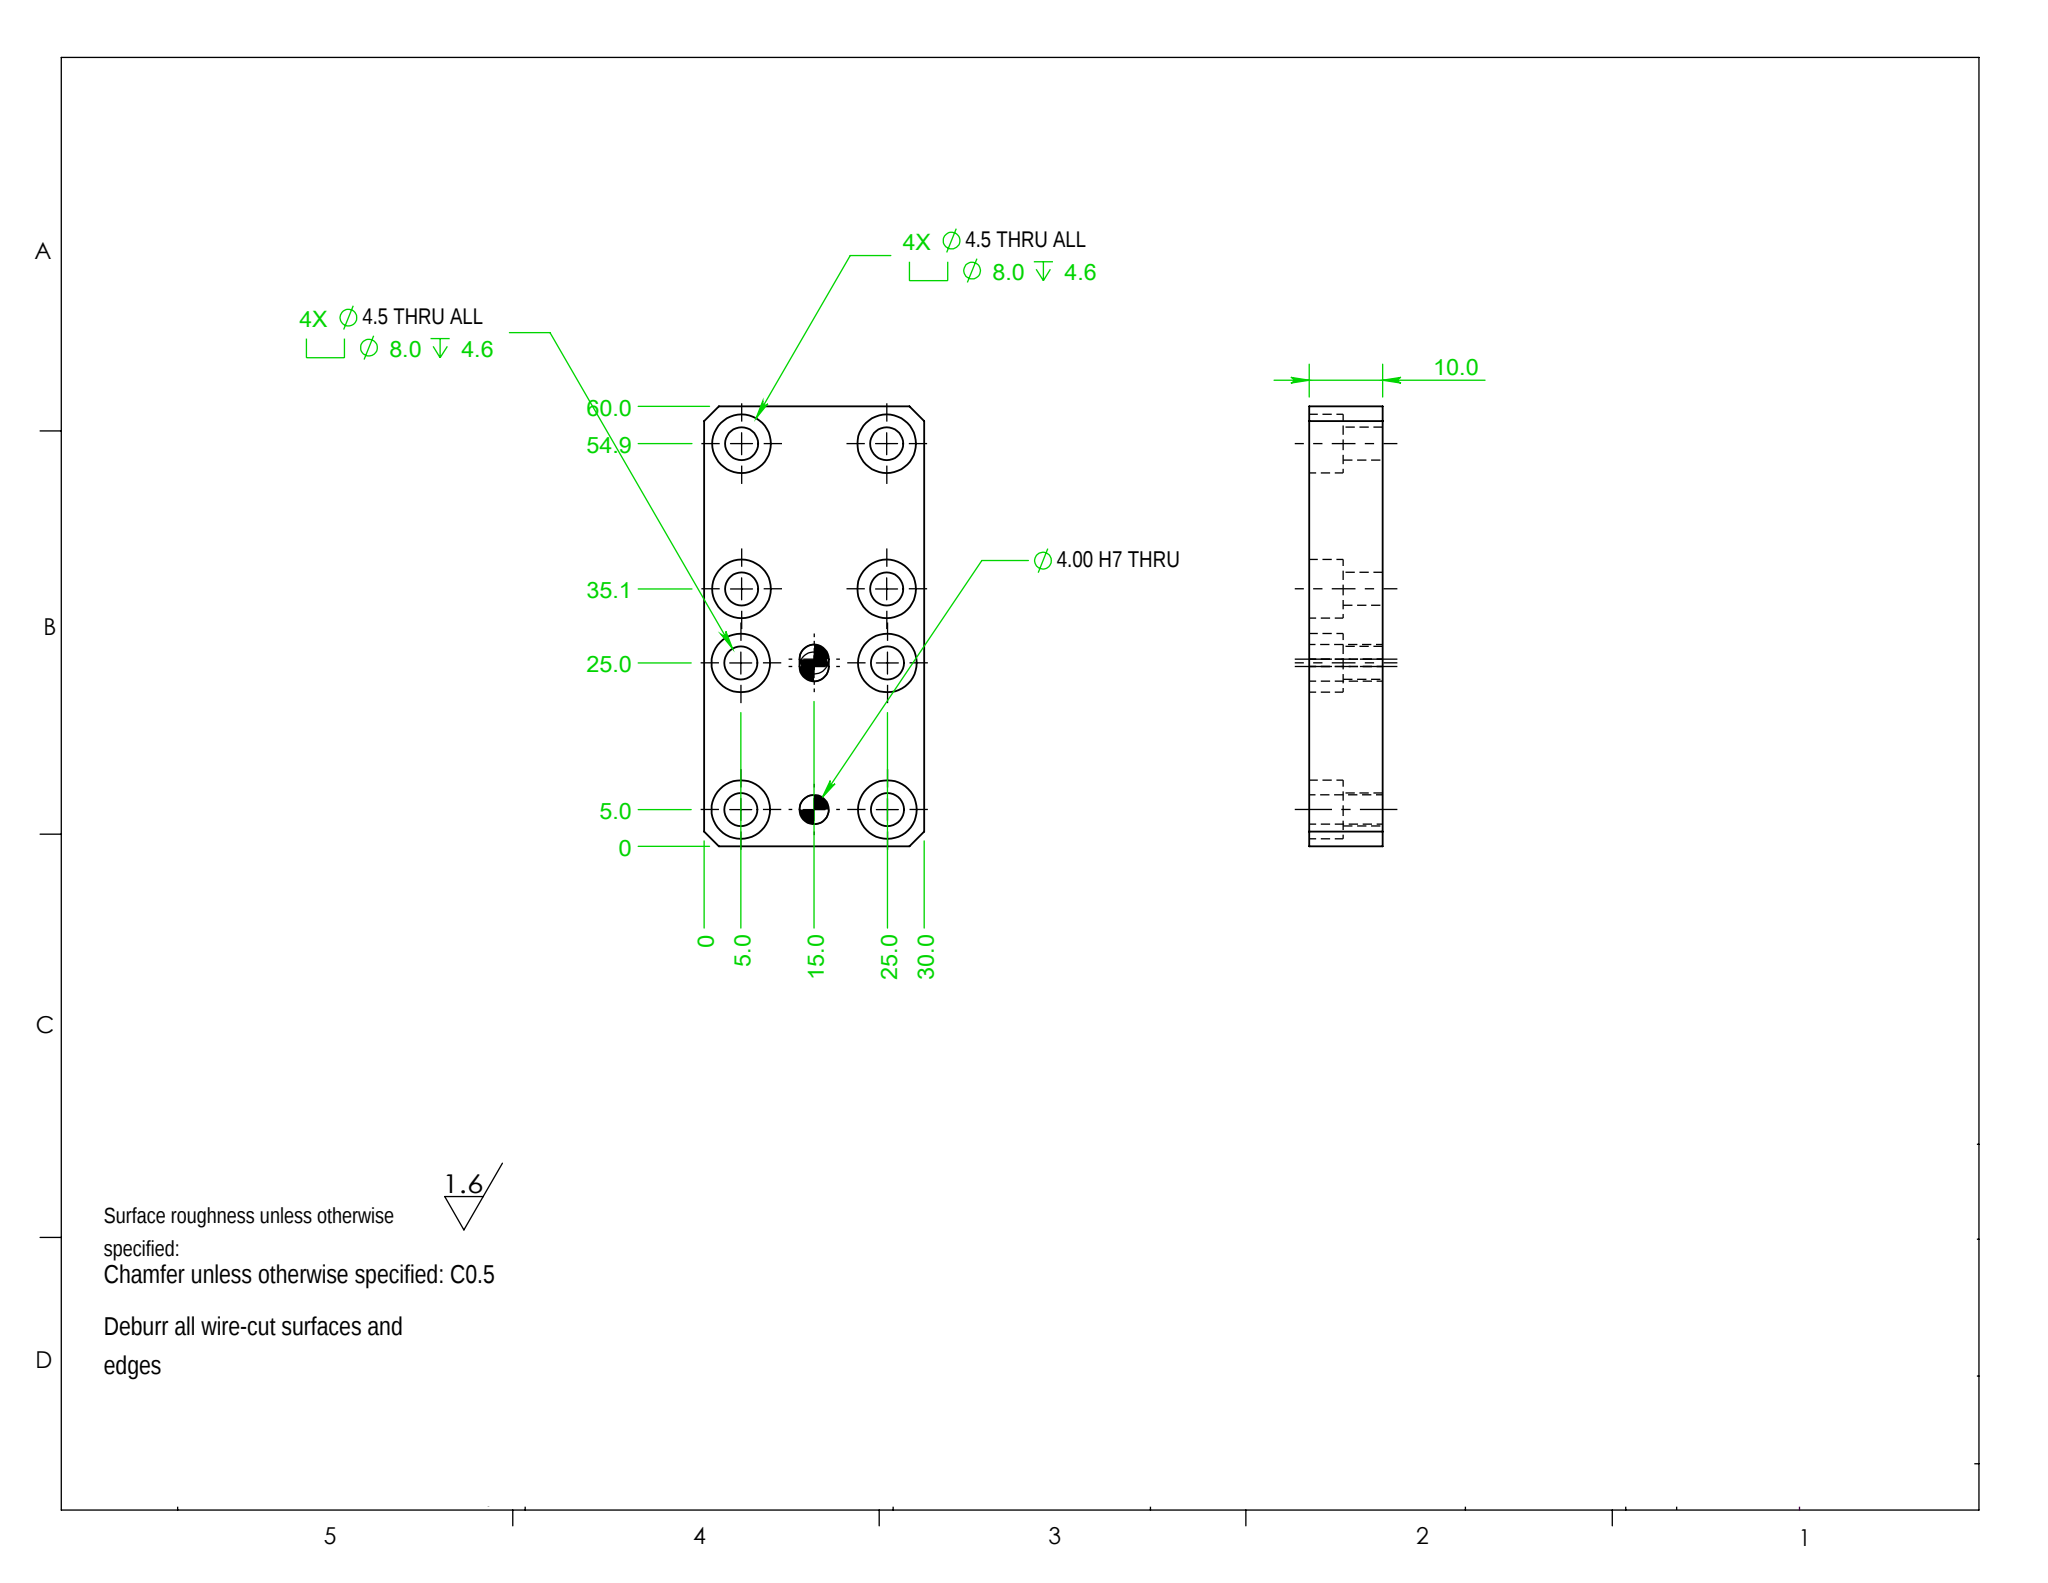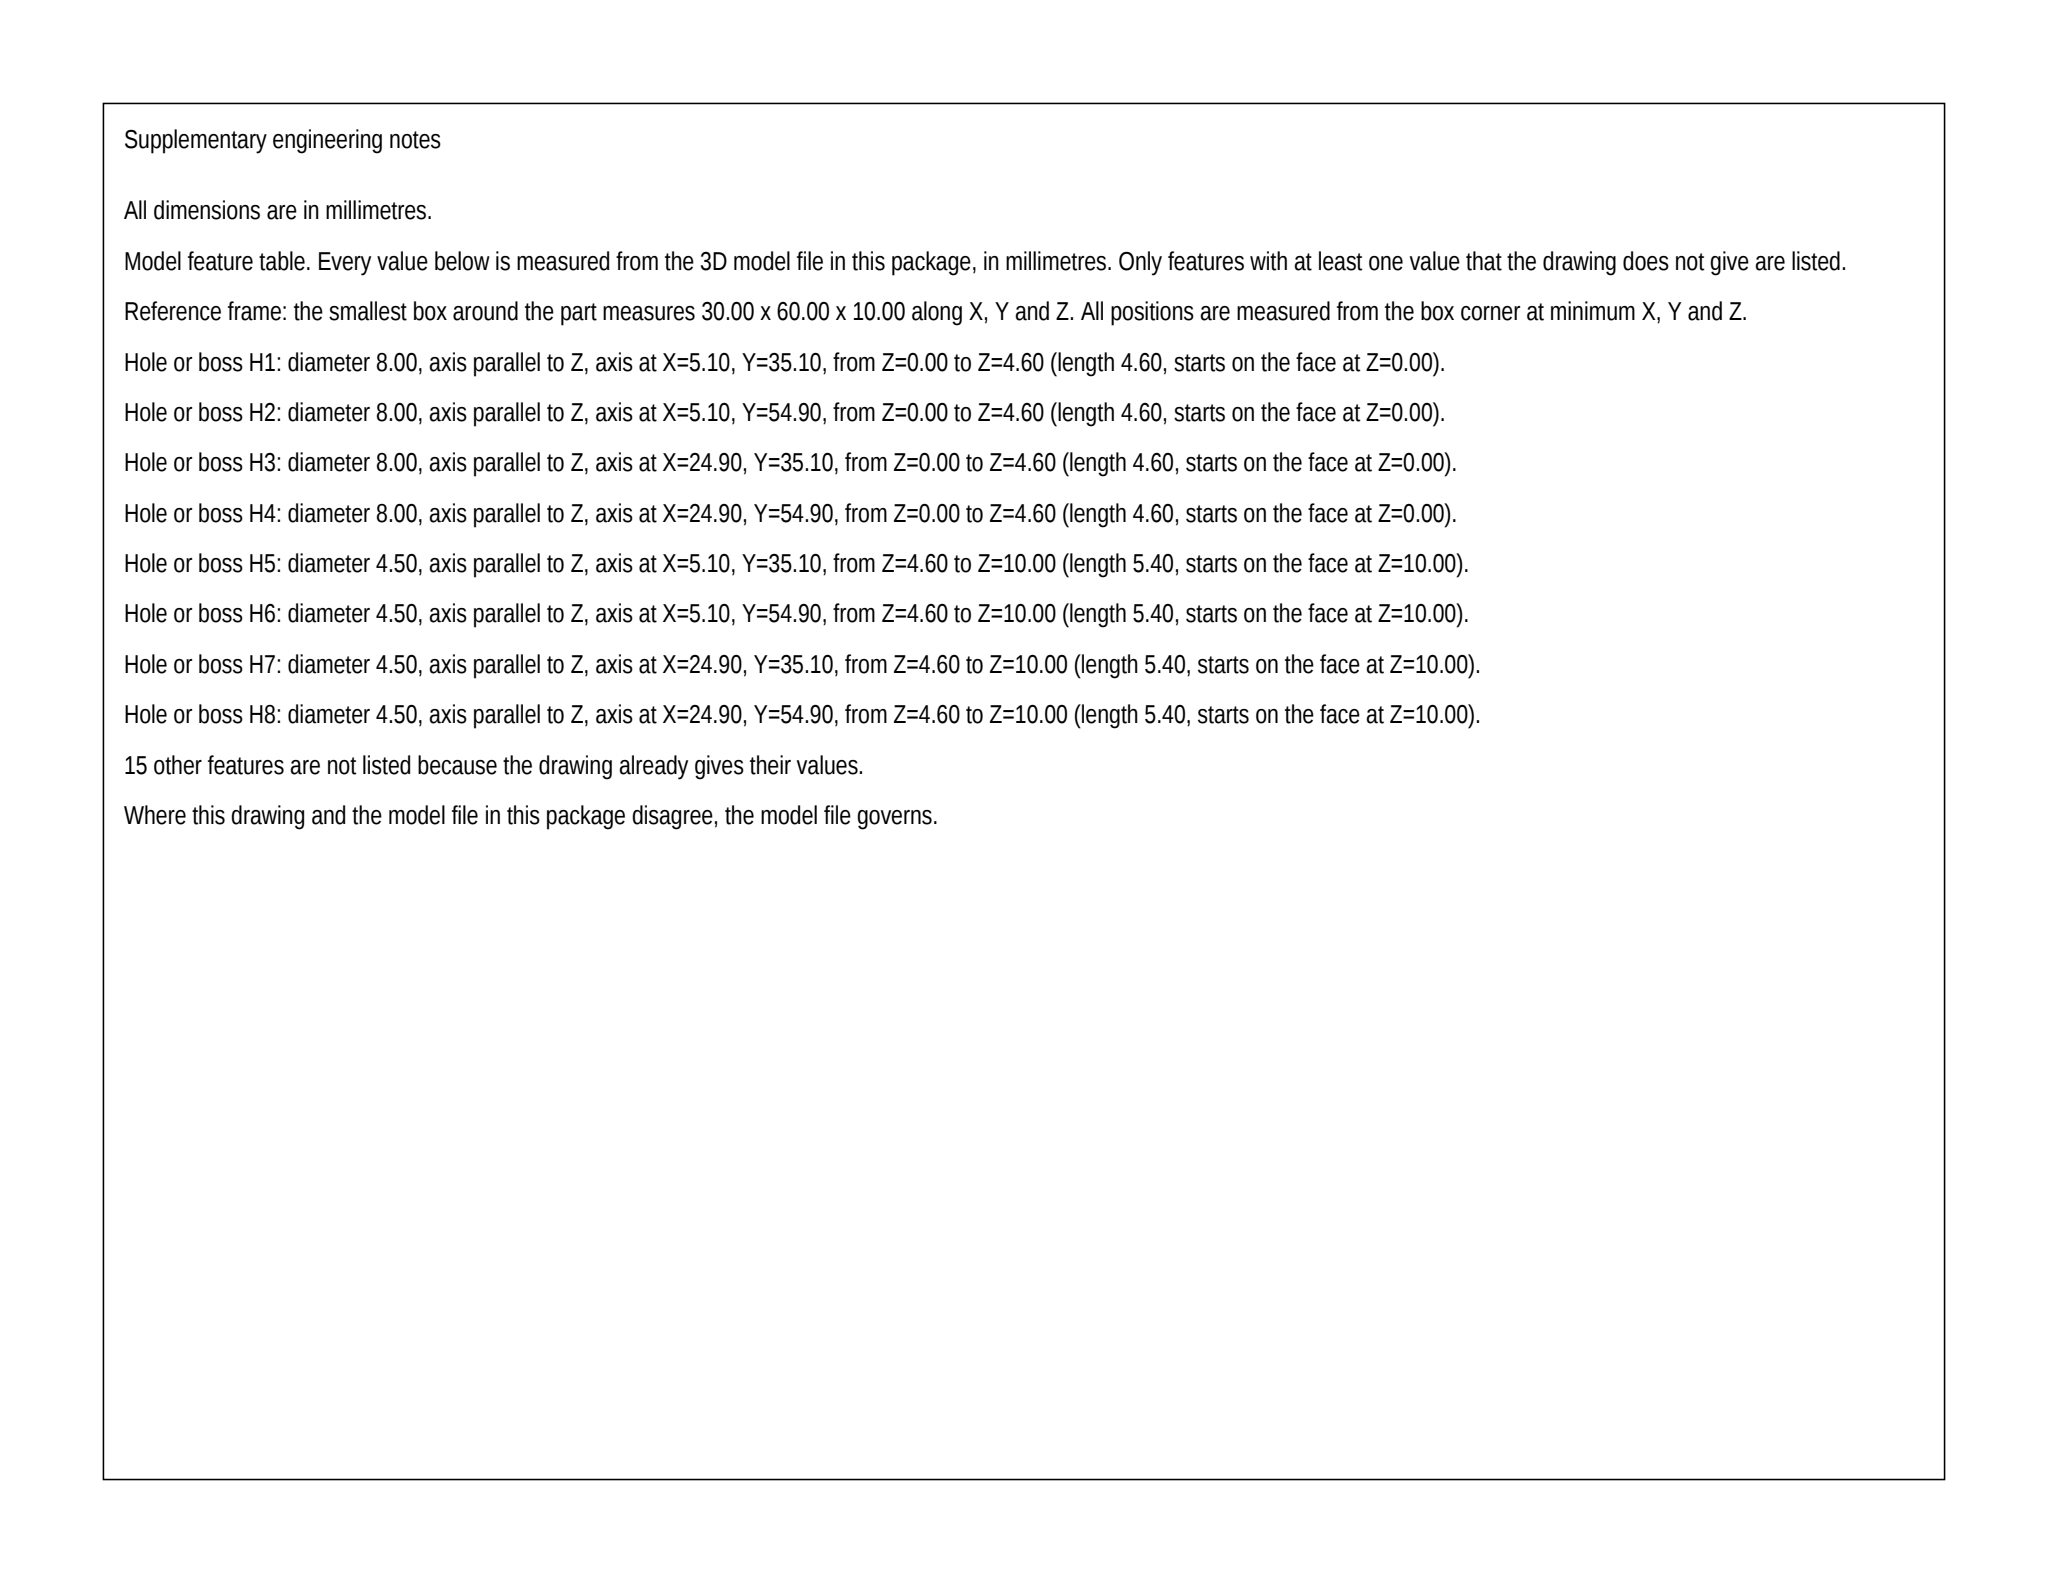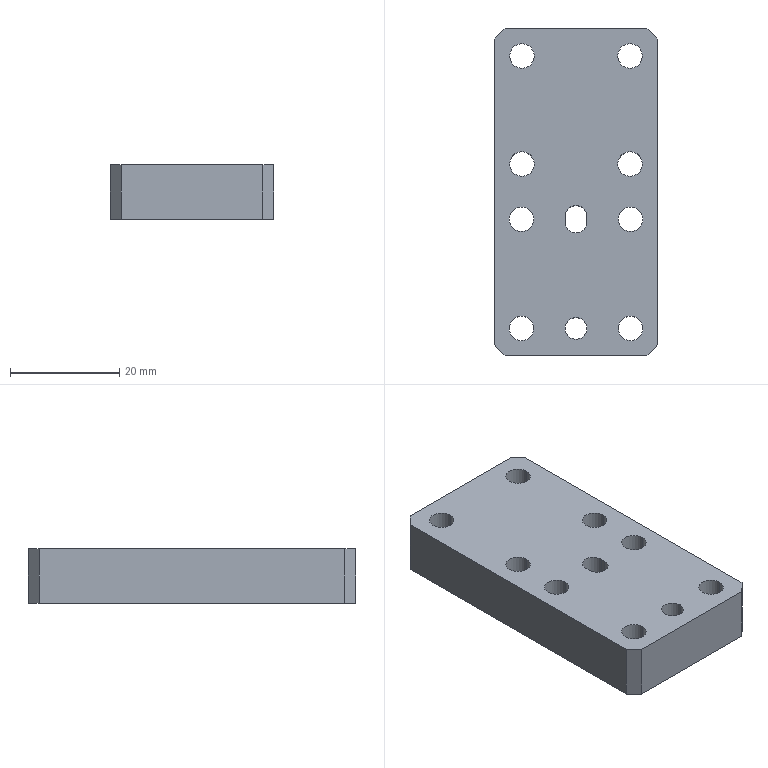Part | SolidWorks | mm | 1 solid | 56 faces | box 30 x 60 x 10 mm | volume 15092 mm3 | cylinder 36 | plane 20 | commonest cylinder face diameters 8 x16 4.5 x16 4 x4
Drawing notes:
4X Ø4.5 THROUGH, CBORE Ø8.0 DP 4.6 (COUNTERBORE) | from the solid: Ø4.5 thru-holes (5.4 deep) each coaxial with Ø8.0 x 4.6 deep bore, z-planes at 4.6; 8 total pairs = 2 notes of 4X
HOLE ROWS Y35.1 & Y54.9: CBORE HOLES AT X5.1 & X24.9 | from the solid: Ø4.5/Ø8.0 cylinders at (5.1,35.1),(24.9,35.1),(5.1,54.9),(24.9,54.9)
4.00 X 5.00 SLOT THRU CTR AT X15.0, Y25.0 | from the solid: Ø4.0 thru cylinders at (15.0,24.5) & (15.0,25.5), slot ctr Y=25.0
TOP HOLE ROW AT Y = 54.9 FROM BOTTOM EDGE | from the solid: Ø4.5 holes at y=54.9; bbox y 0 to 60.0
build123d program:
from build123d import *

# Parameters (mm, degrees)
SKETCH1_W                                         = 30
SKETCH1_H                                         = 60
BOSS_EXTRUDE1_DEPTH                               = 10
HOLE_SIZE_ACCORDING_TO_HEXAGON_SOCKET_D           = 4.5
HOLE_SIZE_ACCORDING_TO_HEXAGON_SOCKET_CBORE_D     = 8
HOLE_SIZE_ACCORDING_TO_HEXAGON_SOCKET_CBORE_DEPTH = 4.6
HOLE_SIZE_ACCORDING_TO_HEXAGON_SO_2_D             = 4.5
HOLE_SIZE_ACCORDING_TO_HEXAGON_SO_2_CBORE_D       = 8
HOLE_SIZE_ACCORDING_TO_HEXAGON_SO_2_CBORE_DEPTH   = 4.6
SKETCH8_R                                         = 2
CUT_EXTRUDE2_DEPTH                                = 36
CHAMFER1_SIZE                                     = 2


with BuildPart() as part:
    # Sketch1 → Boss-Extrude1 (new body)
    with BuildSketch(Plane.XY):
        Rectangle(SKETCH1_W, SKETCH1_H)
    extrude(amount=BOSS_EXTRUDE1_DEPTH)

    # Hole Size _ according to_ Hexagon Socket (through all)
    with Locations(Plane(origin=(0, 0, 0), x_dir=(-1, 0, 0), z_dir=(0, 0, -1))):
        with Locations((-10, -5), (10, -5), (10, -25), (-10, -25)):
            CounterBoreHole(HOLE_SIZE_ACCORDING_TO_HEXAGON_SOCKET_D / 2, HOLE_SIZE_ACCORDING_TO_HEXAGON_SOCKET_CBORE_D / 2, HOLE_SIZE_ACCORDING_TO_HEXAGON_SOCKET_CBORE_DEPTH)

    # Hole Size _ according to_ Hexagon So 2 (through all)
    with Locations(Plane(origin=(0, 0, 0), x_dir=(-1, 0, 0), z_dir=(0, 0, -1))):
        with Locations((9.899, 24.899), (-9.899, 5.101), (-9.899, 24.899), (9.899, 5.101)):
            CounterBoreHole(HOLE_SIZE_ACCORDING_TO_HEXAGON_SO_2_D / 2, HOLE_SIZE_ACCORDING_TO_HEXAGON_SO_2_CBORE_D / 2, HOLE_SIZE_ACCORDING_TO_HEXAGON_SO_2_CBORE_DEPTH)

    # Sketch8 → Cut-Extrude2 (cut, through all)
    with BuildSketch(Plane.XY.offset(10)):
        with Locations((0, -25)):
            Circle(SKETCH8_R)
        with BuildLine():
            Line((-2, -5.5), (-2, -4.5))
            ThreePointArc((-2, -4.5), (0, -2.5), (2, -4.5))
            Line((2, -4.5), (2, -5.5))
            ThreePointArc((2, -5.5), (0, -7.5), (-2, -5.5))
        make_face()
    extrude(amount=-CUT_EXTRUDE2_DEPTH, mode=Mode.SUBTRACT)

    # Chamfer1
    chamfer1_edges = [part.edges().sort_by_distance(p)[0] for p in [
        (-15, 30, 5),
        (15, 30, 5),
        (15, -30, 5),
        (-15, -30, 5),
    ]]
    chamfer(chamfer1_edges, length=CHAMFER1_SIZE)


solid = part.part